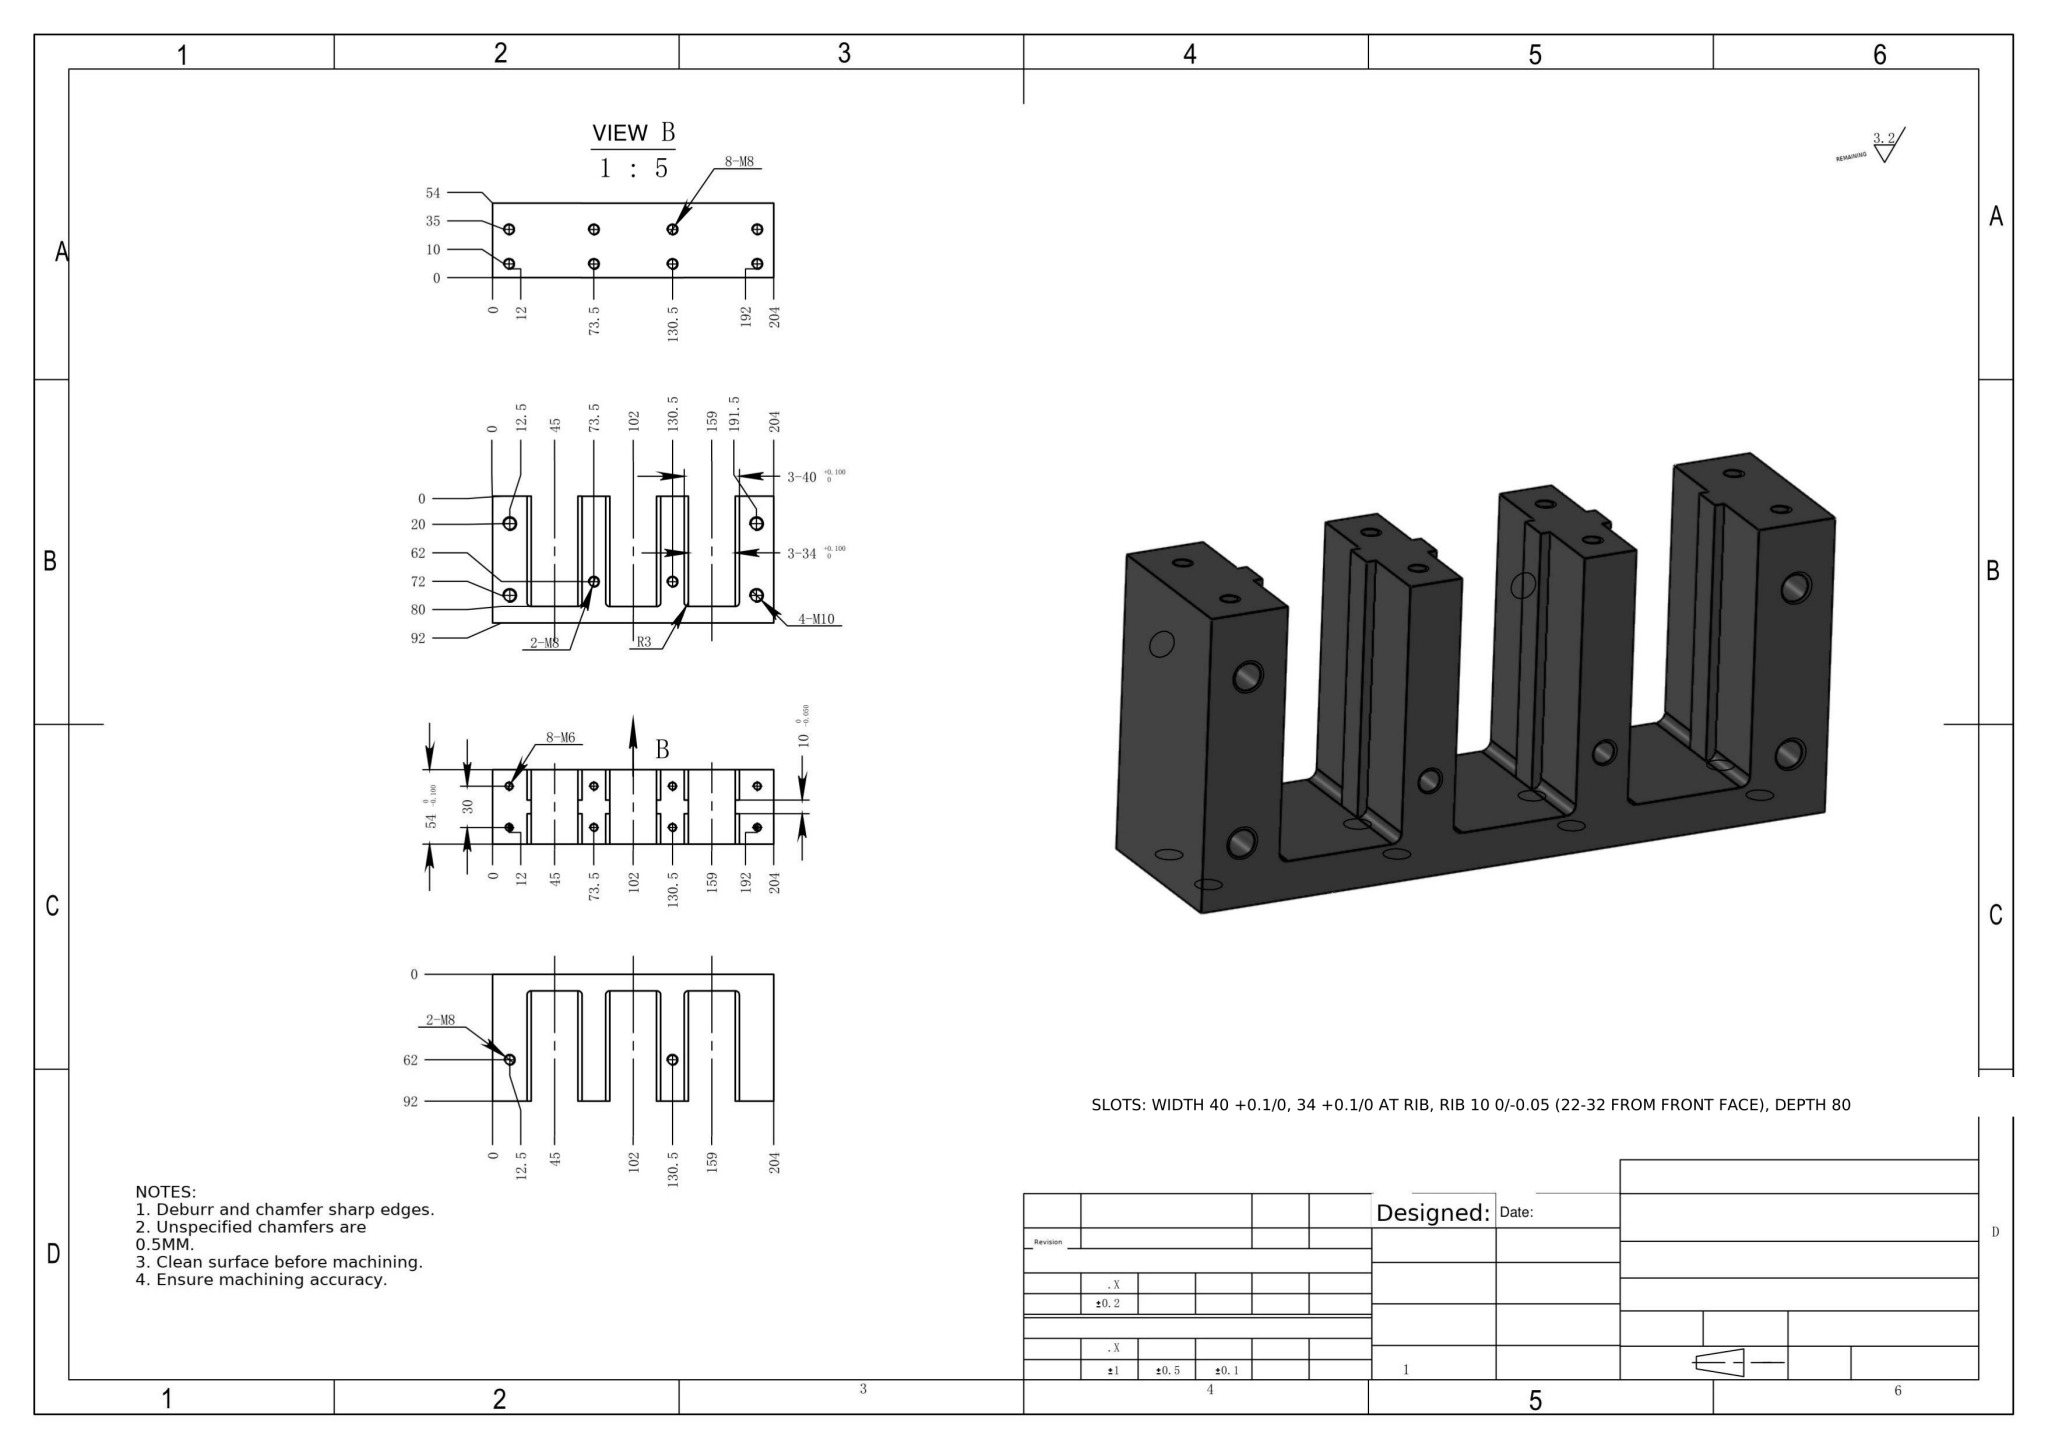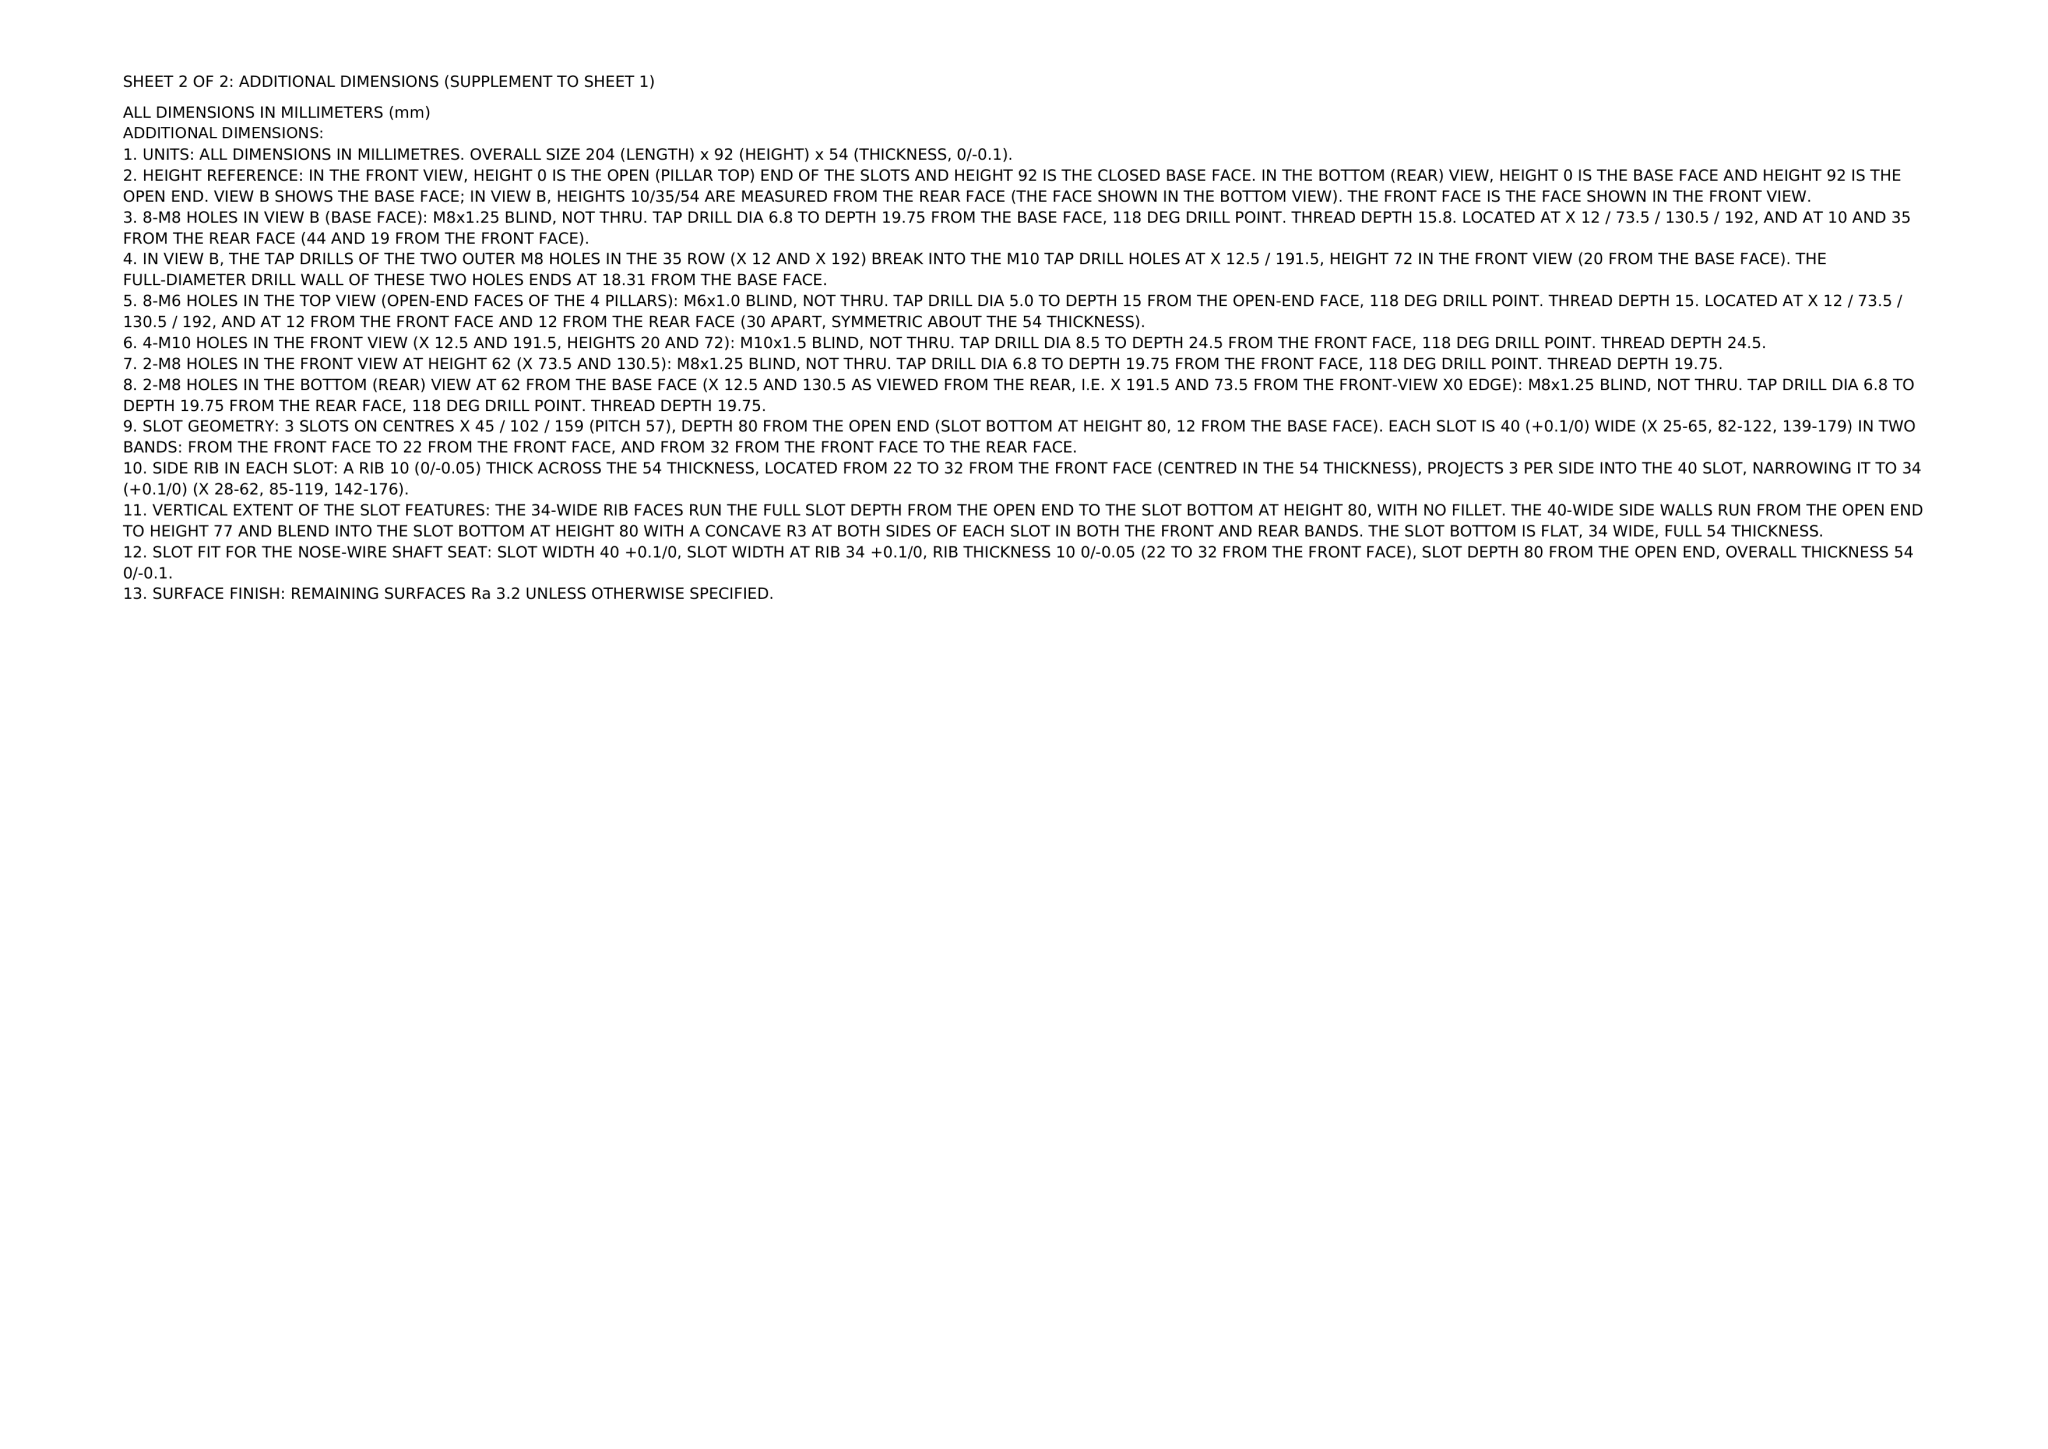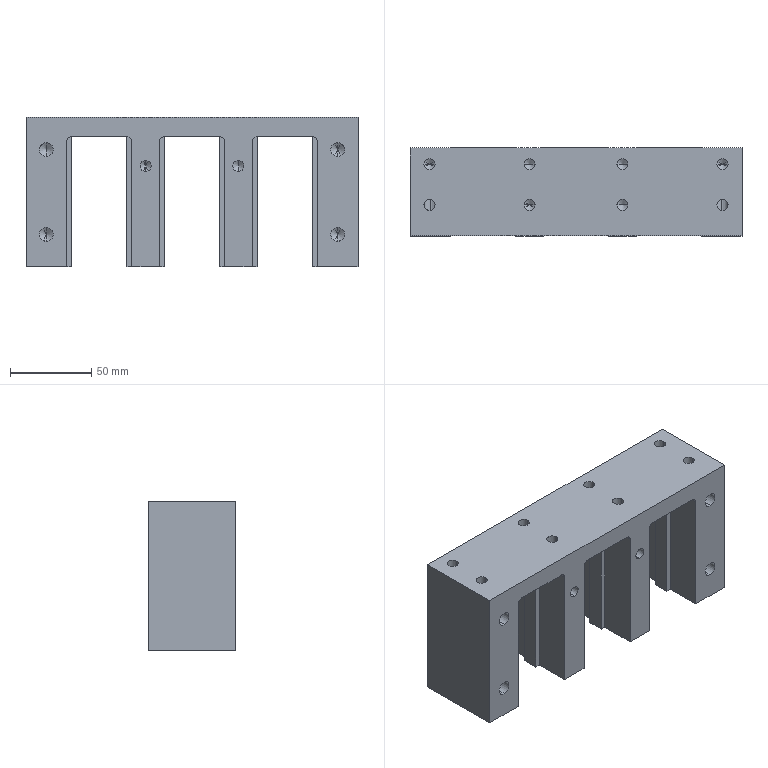Part | NX | mm | 1 solid | 146 faces | box 204 x 54 x 92 mm | volume 493201 mm3 | cylinder 60 | cone 44 | plane 42 | commonest cylinder face diameters 6.8 x24 5 x16 6 x12 8.5 x8